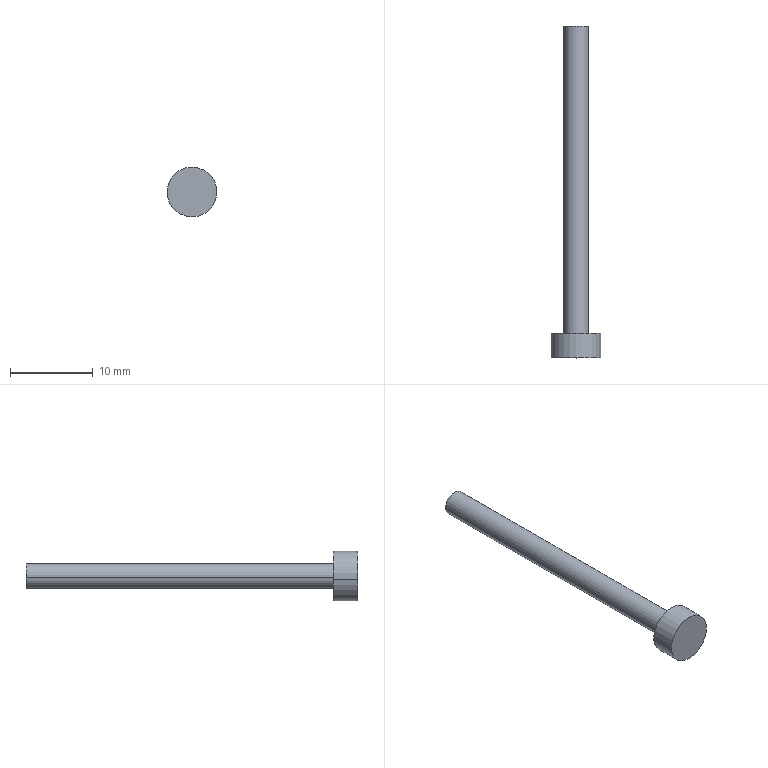Component | SolidWorks | 3mmX34ScrewRod-6 | 1 solid | 7 faces | box 6 x 40 x 6 mm | volume 346 mm3 | cylinder 4 | plane 3 | commonest cylinder face diameters 6 x2 3 x2
build123d program:
from build123d import *

# Parameters (mm, degrees)
SKETCH1_R           = 1.5
BOSS_EXTRUDE1_DEPTH = 18.5
SKETCH2_R           = 3
BOSS_EXTRUDE2_DEPTH = 3


with BuildPart() as part:
    # Sketch1 → Boss-Extrude1 (new, symmetric)
    with BuildSketch(Plane.XY):
        Circle(SKETCH1_R)
    extrude(amount=BOSS_EXTRUDE1_DEPTH, both=True)

    # Sketch2 → Boss-Extrude2 (add)
    with BuildSketch(Plane(origin=(0, 0, -18.5), x_dir=(-1, 0, 0), z_dir=(0, 0, -1))):
        Circle(SKETCH2_R)
    extrude(amount=BOSS_EXTRUDE2_DEPTH)


solid = part.part

# Placed as in the assembly
solid = solid.moved(Location((-16.097, 5.517, 28), (-90, 0, 0)))
STEP:
#1=COLOUR_RGB('',0.7922,0.8196,0.9333);
#2=FILL_AREA_STYLE_COLOUR('',#1);
#3=FILL_AREA_STYLE('',(#2));
#4=SURFACE_STYLE_FILL_AREA(#3);
#5=SURFACE_SIDE_STYLE('',(#4));
#6=SURFACE_STYLE_USAGE(.BOTH.,#5);
#7=PRESENTATION_STYLE_ASSIGNMENT((#6));
#8=CARTESIAN_POINT('',(-0.5166,-0.6292,1.118));
#9=VERTEX_POINT('',#8);
#10=CARTESIAN_POINT('',(-0.7508,-0.6292,1.087));
#11=VERTEX_POINT('',#10);
#12=CARTESIAN_POINT('',(-0.6337,-0.6292,1.102));
#13=DIRECTION('',(0.,-1.,0.));
#14=DIRECTION('',(0.9915,0.,0.1304));
#15=AXIS2_PLACEMENT_3D('',#12,#13,#14);
#16=CIRCLE('',#15,0.1181);
#17=EDGE_CURVE('',#9,#11,#16,.T.);
#18=ORIENTED_EDGE('',*,*,#17,.F.);
#19=CARTESIAN_POINT('',(-0.5166,-0.5111,1.118));
#20=VERTEX_POINT('',#19);
#21=CARTESIAN_POINT('',(-0.5166,-0.6292,1.118));
#22=DIRECTION('',(-0.,1.,-0.));
#23=VECTOR('',#22,39.37);
#24=LINE('',#21,#23);
#25=EDGE_CURVE('',#9,#20,#24,.T.);
#26=ORIENTED_EDGE('',*,*,#25,.T.);
#27=CARTESIAN_POINT('',(-0.7508,-0.5111,1.087));
#28=VERTEX_POINT('',#27);
#29=CARTESIAN_POINT('',(-0.6337,-0.5111,1.102));
#30=DIRECTION('',(0.,-1.,0.));
#31=DIRECTION('',(0.9915,0.,0.1304));
#32=AXIS2_PLACEMENT_3D('',#29,#30,#31);
#33=CIRCLE('',#32,0.1181);
#34=EDGE_CURVE('',#20,#28,#33,.T.);
#35=ORIENTED_EDGE('',*,*,#34,.T.);
#36=CARTESIAN_POINT('',(-0.7508,-0.6292,1.087));
#37=DIRECTION('',(-0.,1.,-0.));
#38=VECTOR('',#37,39.37);
#39=LINE('',#36,#38);
#40=EDGE_CURVE('',#11,#28,#39,.T.);
#41=ORIENTED_EDGE('',*,*,#40,.F.);
#42=EDGE_LOOP('',(#18,#26,#35,#41));
#43=FACE_OUTER_BOUND('',#42,.T.);
#44=CARTESIAN_POINT('',(-0.6337,-0.6292,1.102));
#45=DIRECTION('',(-0.,1.,-0.));
#46=DIRECTION('',(-0.9915,0.,-0.1304));
#47=AXIS2_PLACEMENT_3D('',#44,#45,#46);
#48=CYLINDRICAL_SURFACE('',#47,0.1181);
#49=ADVANCED_FACE('',(#43),#48,.T.);
#50=CARTESIAN_POINT('',(-0.6923,0.9456,1.095));
#51=VERTEX_POINT('',#50);
#52=CARTESIAN_POINT('',(-0.5752,0.9456,1.11));
#53=VERTEX_POINT('',#52);
#54=CARTESIAN_POINT('',(-0.6337,0.9456,1.102));
#55=DIRECTION('',(-0.,1.,-0.));
#56=DIRECTION('',(-0.9915,0.,-0.1304));
#57=AXIS2_PLACEMENT_3D('',#54,#55,#56);
#58=CIRCLE('',#57,0.05906);
#59=EDGE_CURVE('',#51,#53,#58,.T.);
#60=ORIENTED_EDGE('',*,*,#59,.F.);
#61=CARTESIAN_POINT('',(-0.6923,-0.5111,1.095));
#62=VERTEX_POINT('',#61);
#63=CARTESIAN_POINT('',(-0.6923,0.9456,1.095));
#64=DIRECTION('',(0.,-1.,0.));
#65=VECTOR('',#64,39.37);
#66=LINE('',#63,#65);
#67=EDGE_CURVE('',#51,#62,#66,.T.);
#68=ORIENTED_EDGE('',*,*,#67,.T.);
#69=CARTESIAN_POINT('',(-0.5752,-0.5111,1.11));
#70=VERTEX_POINT('',#69);
#71=CARTESIAN_POINT('',(-0.6337,-0.5111,1.102));
#72=DIRECTION('',(0.,-1.,0.));
#73=DIRECTION('',(0.9915,0.,0.1304));
#74=AXIS2_PLACEMENT_3D('',#71,#72,#73);
#75=CIRCLE('',#74,0.05906);
#76=EDGE_CURVE('',#70,#62,#75,.T.);
#77=ORIENTED_EDGE('',*,*,#76,.F.);
#78=CARTESIAN_POINT('',(-0.5752,0.9456,1.11));
#79=DIRECTION('',(0.,-1.,0.));
#80=VECTOR('',#79,39.37);
#81=LINE('',#78,#80);
#82=EDGE_CURVE('',#53,#70,#81,.T.);
#83=ORIENTED_EDGE('',*,*,#82,.F.);
#84=EDGE_LOOP('',(#60,#68,#77,#83));
#85=FACE_OUTER_BOUND('',#84,.T.);
#86=CARTESIAN_POINT('',(-0.6337,0.9456,1.102));
#87=DIRECTION('',(0.,-1.,0.));
#88=DIRECTION('',(0.9915,0.,0.1304));
#89=AXIS2_PLACEMENT_3D('',#86,#87,#88);
#90=CYLINDRICAL_SURFACE('',#89,0.05906);
#91=ADVANCED_FACE('',(#85),#90,.T.);
#92=ORIENTED_EDGE('',*,*,#67,.F.);
#93=CARTESIAN_POINT('',(-0.6337,0.9456,1.102));
#94=DIRECTION('',(-0.,1.,-0.));
#95=DIRECTION('',(-0.9915,0.,-0.1304));
#96=AXIS2_PLACEMENT_3D('',#93,#94,#95);
#97=CIRCLE('',#96,0.05906);
#98=EDGE_CURVE('',#53,#51,#97,.T.);
#99=ORIENTED_EDGE('',*,*,#98,.F.);
#100=ORIENTED_EDGE('',*,*,#82,.T.);
#101=CARTESIAN_POINT('',(-0.6337,-0.5111,1.102));
#102=DIRECTION('',(0.,-1.,0.));
#103=DIRECTION('',(0.9915,0.,0.1304));
#104=AXIS2_PLACEMENT_3D('',#101,#102,#103);
#105=CIRCLE('',#104,0.05906);
#106=EDGE_CURVE('',#62,#70,#105,.T.);
#107=ORIENTED_EDGE('',*,*,#106,.F.);
#108=EDGE_LOOP('',(#92,#99,#100,#107));
#109=FACE_OUTER_BOUND('',#108,.T.);
#110=CARTESIAN_POINT('',(-0.6337,0.9456,1.102));
#111=DIRECTION('',(0.,-1.,0.));
#112=DIRECTION('',(0.9915,0.,0.1304));
#113=AXIS2_PLACEMENT_3D('',#110,#111,#112);
#114=CYLINDRICAL_SURFACE('',#113,0.05906);
#115=ADVANCED_FACE('',(#109),#114,.T.);
#116=ORIENTED_EDGE('',*,*,#98,.T.);
#117=ORIENTED_EDGE('',*,*,#59,.T.);
#118=EDGE_LOOP('',(#116,#117));
#119=FACE_OUTER_BOUND('',#118,.T.);
#120=CARTESIAN_POINT('',(-0.6337,0.9456,1.102));
#121=DIRECTION('',(-0.,1.,-0.));
#122=DIRECTION('',(-0.9915,-0.,-0.1304));
#123=AXIS2_PLACEMENT_3D('',#120,#121,#122);
#124=PLANE('',#123);
#125=ADVANCED_FACE('',(#119),#124,.T.);
#126=CARTESIAN_POINT('',(-0.6337,-0.5111,1.102));
#127=DIRECTION('',(0.,-1.,0.));
#128=DIRECTION('',(0.9915,0.,0.1304));
#129=AXIS2_PLACEMENT_3D('',#126,#127,#128);
#130=CIRCLE('',#129,0.1181);
#131=EDGE_CURVE('',#28,#20,#130,.T.);
#132=ORIENTED_EDGE('',*,*,#131,.F.);
#133=ORIENTED_EDGE('',*,*,#34,.F.);
#134=EDGE_LOOP('',(#132,#133));
#135=FACE_OUTER_BOUND('',#134,.T.);
#136=ORIENTED_EDGE('',*,*,#76,.T.);
#137=ORIENTED_EDGE('',*,*,#106,.T.);
#138=EDGE_LOOP('',(#136,#137));
#139=FACE_BOUND('',#138,.T.);
#140=CARTESIAN_POINT('',(-0.6337,-0.5111,1.102));
#141=DIRECTION('',(0.,-1.,0.));
#142=DIRECTION('',(0.9915,0.,0.1304));
#143=AXIS2_PLACEMENT_3D('',#140,#141,#142);
#144=PLANE('',#143);
#145=ADVANCED_FACE('',(#135,#139),#144,.F.);
#146=ORIENTED_EDGE('',*,*,#25,.F.);
#147=CARTESIAN_POINT('',(-0.6337,-0.6292,1.102));
#148=DIRECTION('',(0.,-1.,0.));
#149=DIRECTION('',(0.9915,0.,0.1304));
#150=AXIS2_PLACEMENT_3D('',#147,#148,#149);
#151=CIRCLE('',#150,0.1181);
#152=EDGE_CURVE('',#11,#9,#151,.T.);
#153=ORIENTED_EDGE('',*,*,#152,.F.);
#154=ORIENTED_EDGE('',*,*,#40,.T.);
#155=ORIENTED_EDGE('',*,*,#131,.T.);
#156=EDGE_LOOP('',(#146,#153,#154,#155));
#157=FACE_OUTER_BOUND('',#156,.T.);
#158=CARTESIAN_POINT('',(-0.6337,-0.6292,1.102));
#159=DIRECTION('',(-0.,1.,-0.));
#160=DIRECTION('',(-0.9915,0.,-0.1304));
#161=AXIS2_PLACEMENT_3D('',#158,#159,#160);
#162=CYLINDRICAL_SURFACE('',#161,0.1181);
#163=ADVANCED_FACE('',(#157),#162,.T.);
#164=ORIENTED_EDGE('',*,*,#152,.T.);
#165=ORIENTED_EDGE('',*,*,#17,.T.);
#166=EDGE_LOOP('',(#164,#165));
#167=FACE_OUTER_BOUND('',#166,.T.);
#168=CARTESIAN_POINT('',(-0.6337,-0.6292,1.102));
#169=DIRECTION('',(0.,-1.,0.));
#170=DIRECTION('',(0.9915,0.,0.1304));
#171=AXIS2_PLACEMENT_3D('',#168,#169,#170);
#172=PLANE('',#171);
#173=ADVANCED_FACE('',(#167),#172,.T.);
#174=CLOSED_SHELL('',(#49,#91,#115,#125,#145,#163,#173));
#175=MANIFOLD_SOLID_BREP('',#174);
#176=STYLED_ITEM('',(#7),#175);
#177=PRESENTATION_LAYER_ASSIGNMENT('','',(#176));
#178=CARTESIAN_POINT('',(0.,0.,0.));
#179=DIRECTION('',(0.,0.,1.));
#180=DIRECTION('',(1.,0.,0.));
#181=AXIS2_PLACEMENT_3D('',#178,#179,#180);
#182=(LENGTH_UNIT()NAMED_UNIT(*)SI_UNIT($,.METRE.));
#183=LENGTH_MEASURE_WITH_UNIT(LENGTH_MEASURE(0.0254),#182);
#184=DIMENSIONAL_EXPONENTS(1.,0.,0.,0.,0.,0.,0.);
#185=(CONVERSION_BASED_UNIT('',#183)LENGTH_UNIT()NAMED_UNIT(#184));
#186=UNCERTAINTY_MEASURE_WITH_UNIT(LENGTH_MEASURE(0.00001),#185,'','');
#187=(NAMED_UNIT(*)PLANE_ANGLE_UNIT()SI_UNIT($,.RADIAN.));
#188=(NAMED_UNIT(*)SI_UNIT($,.STERADIAN.)SOLID_ANGLE_UNIT());
#189=(GEOMETRIC_REPRESENTATION_CONTEXT(3)GLOBAL_UNCERTAINTY_ASSIGNED_CONTEXT((#186))GLOBAL_UNIT_ASSIGNED_CONTEXT((#185,#187,#188))REPRESENTATION_CONTEXT('',''));
#190=ADVANCED_BREP_SHAPE_REPRESENTATION('',(#175,#181),#189);
#191=(LENGTH_UNIT()NAMED_UNIT(*)SI_UNIT($,.METRE.));
#192=LENGTH_MEASURE_WITH_UNIT(LENGTH_MEASURE(0.0254),#191);
#193=DIMENSIONAL_EXPONENTS(1.,0.,0.,0.,0.,0.,0.);
#194=(CONVERSION_BASED_UNIT('',#192)LENGTH_UNIT()NAMED_UNIT(#193));
#195=UNCERTAINTY_MEASURE_WITH_UNIT(LENGTH_MEASURE(0.00001),#194,'','');
#196=(NAMED_UNIT(*)PLANE_ANGLE_UNIT()SI_UNIT($,.RADIAN.));
#197=(NAMED_UNIT(*)SI_UNIT($,.STERADIAN.)SOLID_ANGLE_UNIT());
#198=(GEOMETRIC_REPRESENTATION_CONTEXT(3)GLOBAL_UNCERTAINTY_ASSIGNED_CONTEXT((#195))GLOBAL_UNIT_ASSIGNED_CONTEXT((#194,#196,#197))REPRESENTATION_CONTEXT('',''));
#199=MECHANICAL_DESIGN_GEOMETRIC_PRESENTATION_REPRESENTATION('',(#176),#198);